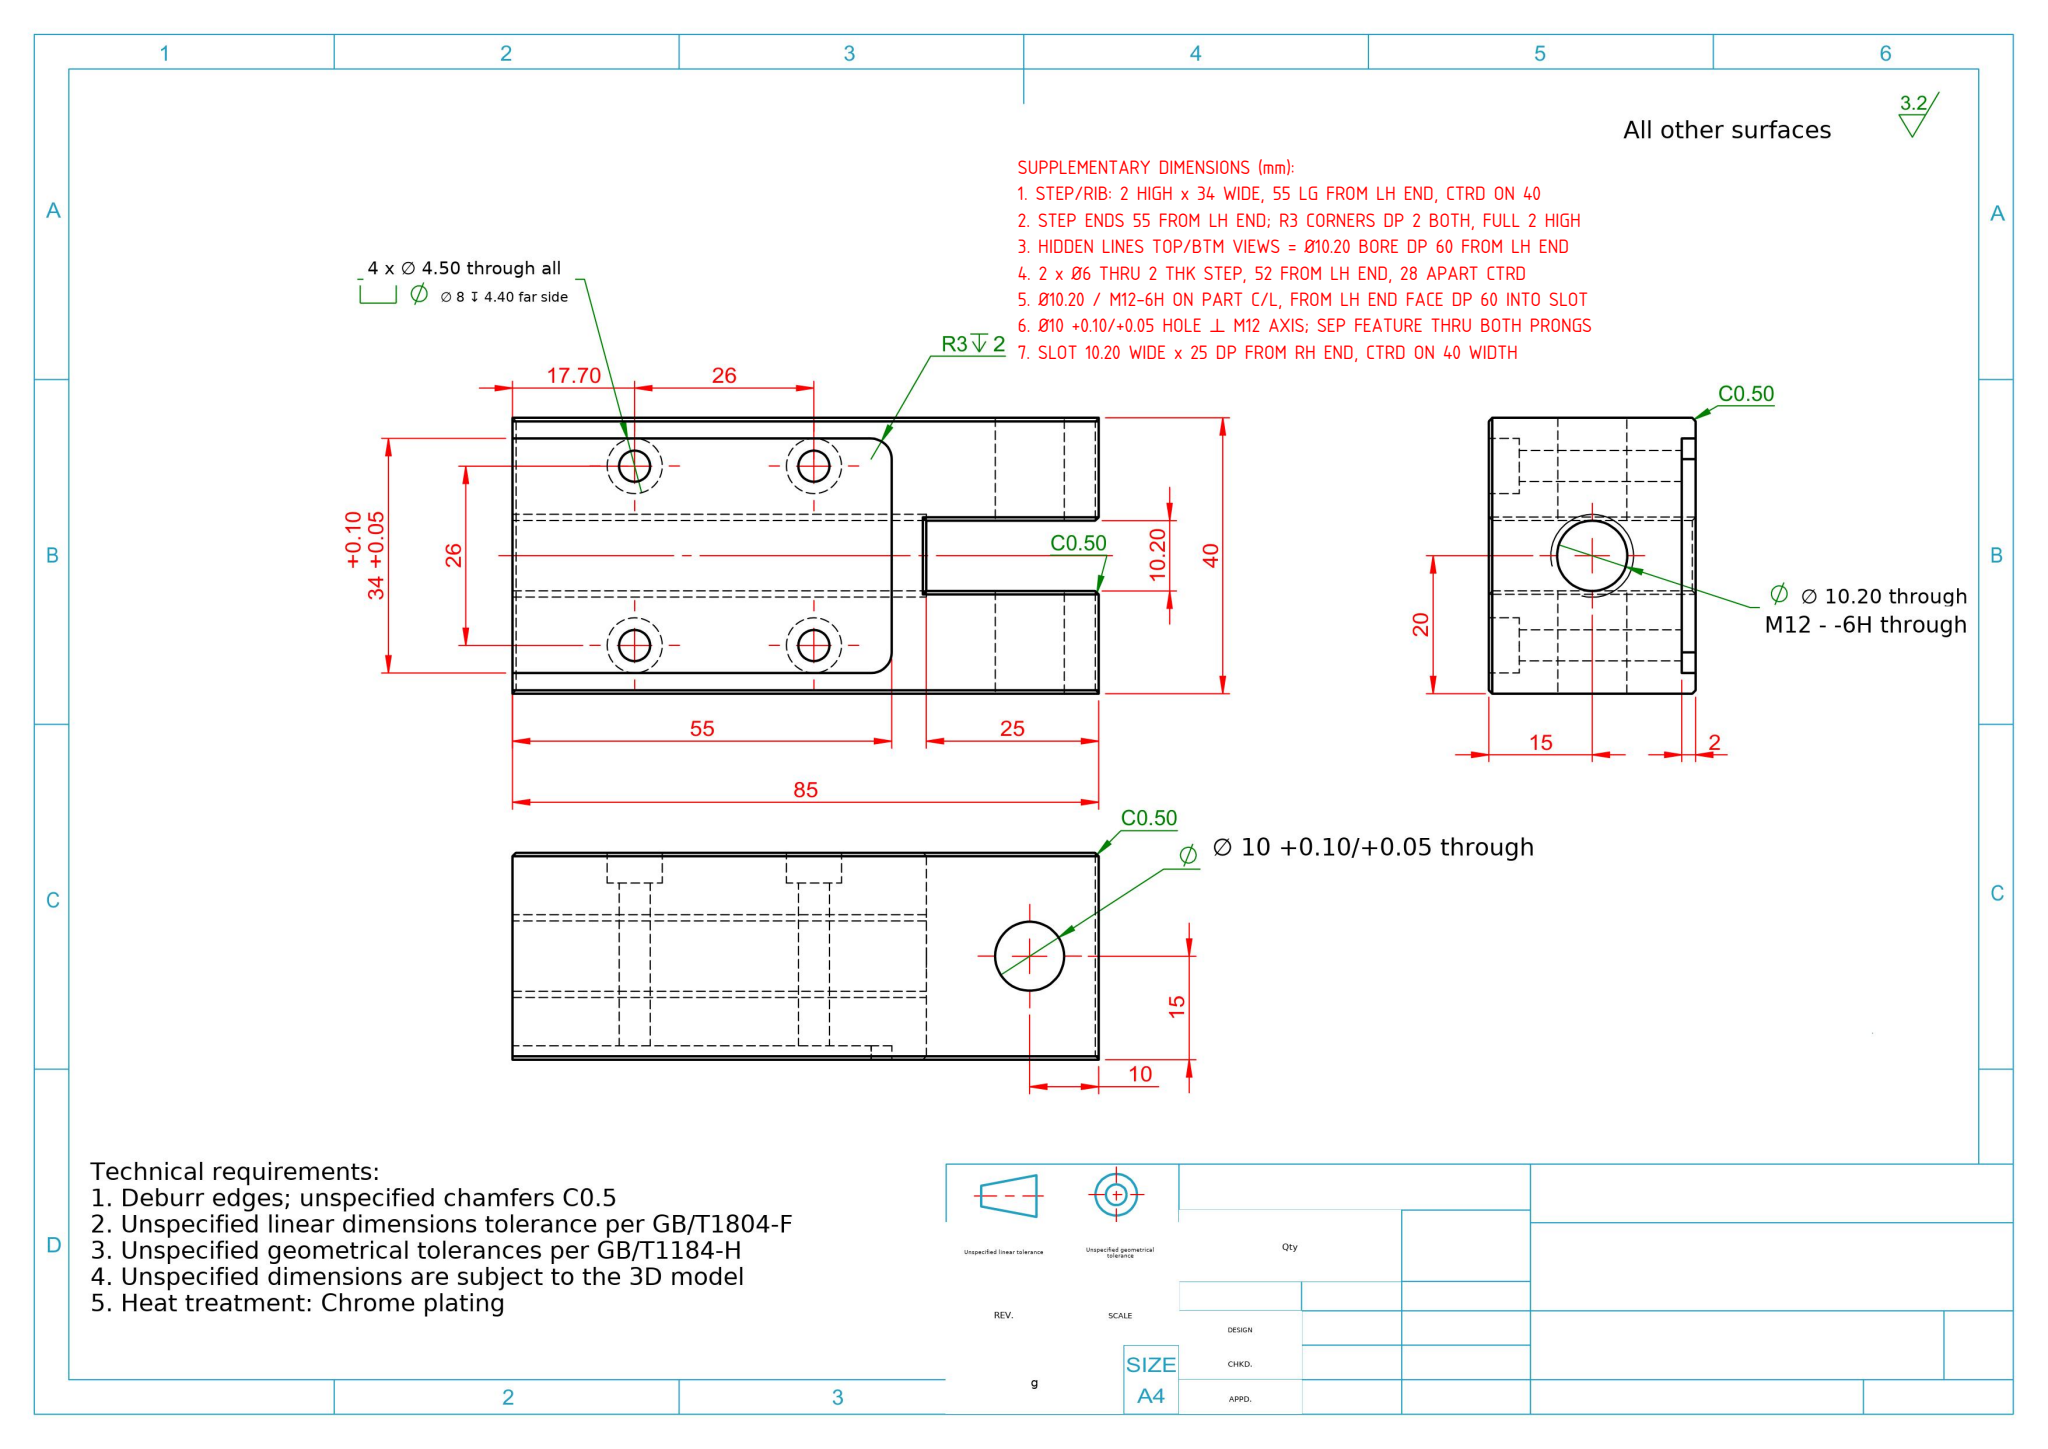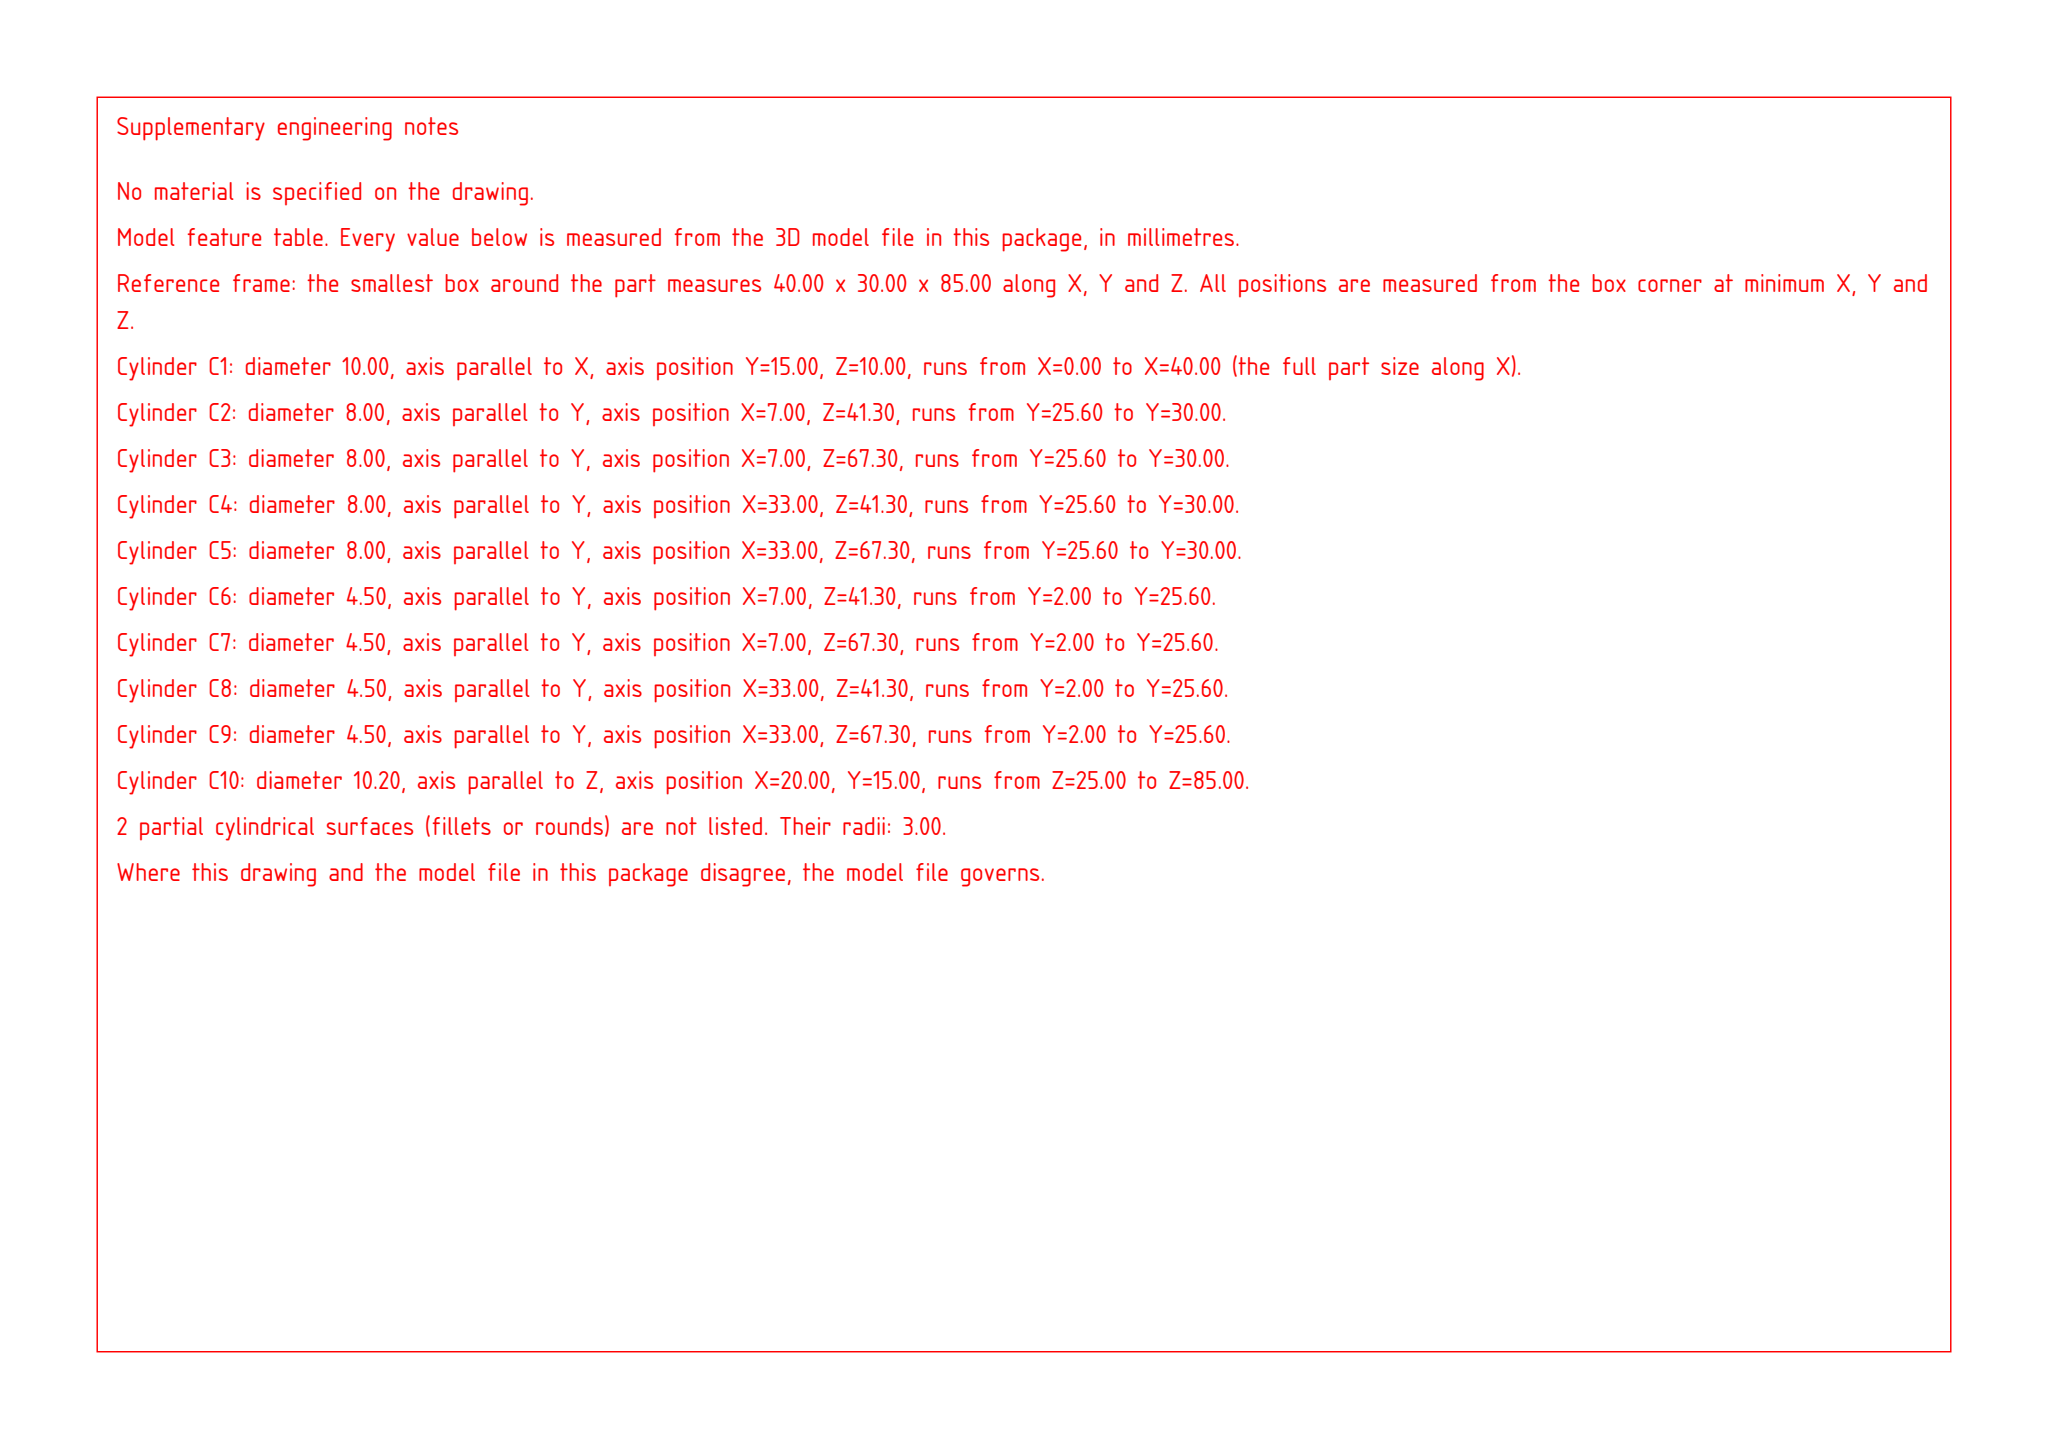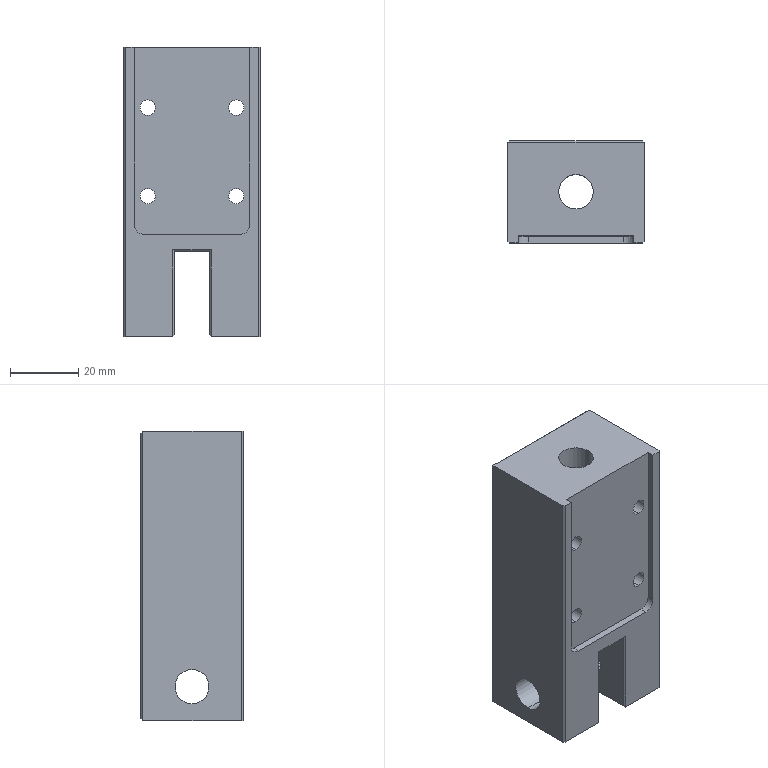Part | SolidWorks | mm | 1 solid | 60 faces | box 40 x 30 x 85 mm | volume 80915 mm3 | plane 36 | cylinder 24 | commonest cylinder face diameters 8 x8 4.5 x8 10 x4 10.2 x2 6 x2
build123d program:
from build123d import *

# Parameters (mm, degrees)
SKETCH1_W                                       = 40
SKETCH1_H                                       = 30
BOSS_EXTRUDE1_DEPTH                             = 85
SKETCH4_W                                       = 10.2
SKETCH4_H                                       = 30
CUT_EXTRUDE3_DEPTH                              = 25
SKETCH5_R                                       = 5
CUT_EXTRUDE4_DEPTH                              = 96.131
M12_TAPPED_HOLE1_D                              = 10.2
SKETCH13_W                                      = 34
SKETCH13_H                                      = 55
CUT_EXTRUDE6_DEPTH                              = 2
FILLET3_R                                       = 3
M4_HEX_SOCKET_HEAD_CAP_SCREW_CBORE1_D           = 4.5
M4_HEX_SOCKET_HEAD_CAP_SCREW_CBORE1_CBORE_D     = 8
M4_HEX_SOCKET_HEAD_CAP_SCREW_CBORE1_CBORE_DEPTH = 4.4
CHAMFER1_SIZE                                   = 0.5


with BuildPart() as part:
    # Sketch1 → Boss-Extrude1 (new body)
    with BuildSketch(Plane.XY):
        Rectangle(SKETCH1_W, SKETCH1_H)
    extrude(amount=BOSS_EXTRUDE1_DEPTH)

    # Sketch4 → Cut-Extrude3 (cut)
    with BuildSketch(Plane(origin=(0, 0, 0), x_dir=(-1, 0, 0), z_dir=(0, 0, -1))):
        Rectangle(SKETCH4_W, SKETCH4_H)
    extrude(amount=-CUT_EXTRUDE3_DEPTH, mode=Mode.SUBTRACT)

    # Sketch5 → Cut-Extrude4 (cut, through all)
    with BuildSketch(Plane.ZY.offset(20)):
        with Locations((10, 0)):
            Circle(SKETCH5_R)
    extrude(amount=-CUT_EXTRUDE4_DEPTH, mode=Mode.SUBTRACT)

    # M12 Tapped Hole1 (through all)
    with Locations(Plane.XY.offset(85)):
        with Locations((0, 0)):
            Hole(M12_TAPPED_HOLE1_D / 2)

    # Sketch13 → Cut-Extrude6 (cut)
    with BuildSketch(Plane(origin=(0, -15, 0), x_dir=(1, 0, 0), z_dir=(0, 1, 0))):
        with Locations((0, -57.5)):
            Rectangle(SKETCH13_W, SKETCH13_H)
    extrude(amount=CUT_EXTRUDE6_DEPTH, mode=Mode.SUBTRACT)

    # Fillet3
    fillet3_edges = [part.edges().sort_by_distance(p)[0] for p in [
        (-17, -14, 30),
        (17, -14, 30),
    ]]
    fillet(fillet3_edges, radius=FILLET3_R)

    # M4 Hex Socket Head Cap Screw CBORE1 (through all)
    with Locations(Plane(origin=(0, 15, 0), x_dir=(1, 0, 0), z_dir=(0, 1, 0))):
        with Locations((-13, -41.3), (-13, -67.3), (13, -67.3), (13, -41.3)):
            CounterBoreHole(M4_HEX_SOCKET_HEAD_CAP_SCREW_CBORE1_D / 2, M4_HEX_SOCKET_HEAD_CAP_SCREW_CBORE1_CBORE_D / 2, M4_HEX_SOCKET_HEAD_CAP_SCREW_CBORE1_CBORE_DEPTH)

    # Chamfer1
    chamfer1_edges = [part.edges().sort_by_distance(p)[0] for p in [
        (-20, -15, 42.5),
        (0, 15, 85),
        (5.1, 0, 0),
        (5.1, -15, 12.5),
        (0, -15, 25),
        (-5.1, -15, 12.5),
        (-5.1, 0, 0),
        (-20, 15, 42.5),
        (-12.55, 15, 0),
        (-5.1, 15, 12.5),
        (0, 15, 25),
        (5.1, 15, 12.5),
        (12.55, 15, 0),
        (20, 15, 42.5),
        (20, -15, 42.5),
    ]]
    chamfer(chamfer1_edges, length=CHAMFER1_SIZE)


solid = part.part